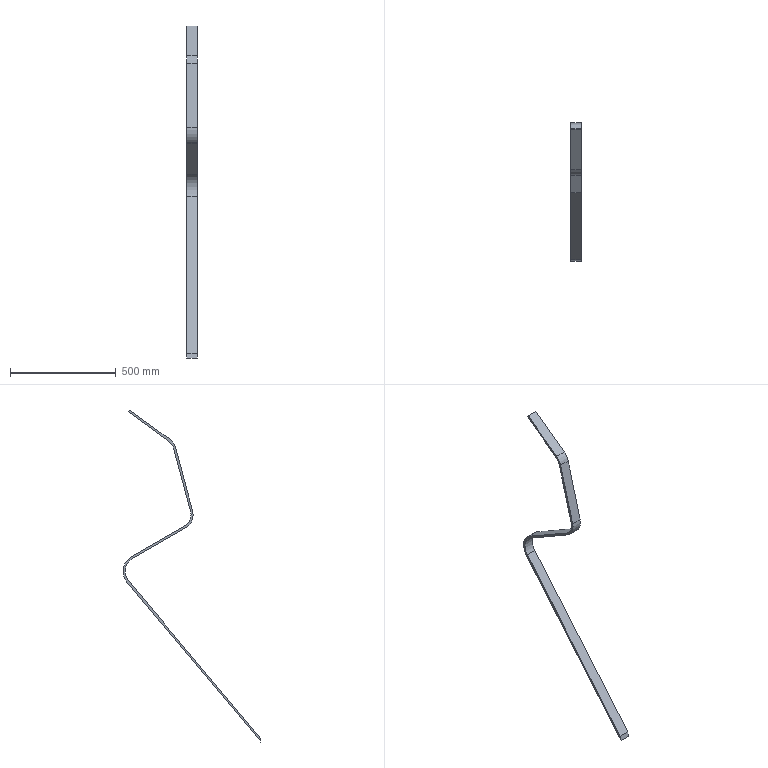Component | SolidWorks | Sipka resetke-1 | 1 solid | 20 faces | box 50 x 651.53 x 1567.49 mm | volume 1035206 mm3 | plane 12 | cylinder 8 | commonest cylinder face diameters 140 x4 120 x3 160 x1
STEP:
#1=COLOUR_RGB('',0.7922,0.8196,0.9333);
#2=FILL_AREA_STYLE_COLOUR('',#1);
#3=FILL_AREA_STYLE('',(#2));
#4=SURFACE_STYLE_FILL_AREA(#3);
#5=SURFACE_SIDE_STYLE('',(#4));
#6=SURFACE_STYLE_USAGE(.BOTH.,#5);
#7=PRESENTATION_STYLE_ASSIGNMENT((#6));
#8=CARTESIAN_POINT('',(-0.1417,16.681,-14.25));
#9=VERTEX_POINT('',#8);
#10=CARTESIAN_POINT('',(-0.1417,16.343,-14.014));
#11=VERTEX_POINT('',#10);
#12=CARTESIAN_POINT('',(-0.1417,17.861,-12.204));
#13=DIRECTION('',(-1.,0.,0.));
#14=DIRECTION('',(0.,0.6427,0.7661));
#15=AXIS2_PLACEMENT_3D('',#12,#13,#14);
#16=CIRCLE('',#15,2.362);
#17=EDGE_CURVE('',#9,#11,#16,.T.);
#18=ORIENTED_EDGE('',*,*,#17,.T.);
#19=CARTESIAN_POINT('',(1.827,16.343,-14.014));
#20=VERTEX_POINT('',#19);
#21=CARTESIAN_POINT('',(-0.1417,16.343,-14.014));
#22=DIRECTION('',(1.,-0.,-0.));
#23=VECTOR('',#22,39.37);
#24=LINE('',#21,#23);
#25=EDGE_CURVE('',#11,#20,#24,.T.);
#26=ORIENTED_EDGE('',*,*,#25,.T.);
#27=CARTESIAN_POINT('',(1.827,16.681,-14.25));
#28=VERTEX_POINT('',#27);
#29=CARTESIAN_POINT('',(1.827,17.861,-12.204));
#30=DIRECTION('',(-1.,0.,0.));
#31=DIRECTION('',(0.,0.6427,0.7661));
#32=AXIS2_PLACEMENT_3D('',#29,#30,#31);
#33=CIRCLE('',#32,2.362);
#34=EDGE_CURVE('',#28,#20,#33,.T.);
#35=ORIENTED_EDGE('',*,*,#34,.F.);
#36=CARTESIAN_POINT('',(-0.1417,16.681,-14.25));
#37=DIRECTION('',(1.,-0.,-0.));
#38=VECTOR('',#37,39.37);
#39=LINE('',#36,#38);
#40=EDGE_CURVE('',#9,#28,#39,.T.);
#41=ORIENTED_EDGE('',*,*,#40,.F.);
#42=EDGE_LOOP('',(#18,#26,#35,#41));
#43=FACE_OUTER_BOUND('',#42,.T.);
#44=CARTESIAN_POINT('',(-0.1417,17.861,-12.204));
#45=DIRECTION('',(1.,-0.,-0.));
#46=DIRECTION('',(-0.,-0.6427,-0.7661));
#47=AXIS2_PLACEMENT_3D('',#44,#45,#46);
#48=CYLINDRICAL_SURFACE('',#47,2.362);
#49=ADVANCED_FACE('',(#43),#48,.F.);
#50=CARTESIAN_POINT('',(-0.1417,15.199,-11.491));
#51=VERTEX_POINT('',#50);
#52=CARTESIAN_POINT('',(-0.1417,16.09,-14.315));
#53=VERTEX_POINT('',#52);
#54=CARTESIAN_POINT('',(-0.1417,17.861,-12.204));
#55=DIRECTION('',(1.,-0.,-0.));
#56=DIRECTION('',(0.,0.6427,0.7661));
#57=AXIS2_PLACEMENT_3D('',#54,#55,#56);
#58=CIRCLE('',#57,2.756);
#59=EDGE_CURVE('',#51,#53,#58,.T.);
#60=ORIENTED_EDGE('',*,*,#59,.T.);
#61=CARTESIAN_POINT('',(1.827,16.09,-14.315));
#62=VERTEX_POINT('',#61);
#63=CARTESIAN_POINT('',(-0.1417,16.09,-14.315));
#64=DIRECTION('',(1.,-0.,-0.));
#65=VECTOR('',#64,39.37);
#66=LINE('',#63,#65);
#67=EDGE_CURVE('',#53,#62,#66,.T.);
#68=ORIENTED_EDGE('',*,*,#67,.T.);
#69=CARTESIAN_POINT('',(1.827,15.199,-11.491));
#70=VERTEX_POINT('',#69);
#71=CARTESIAN_POINT('',(1.827,17.861,-12.204));
#72=DIRECTION('',(1.,-0.,-0.));
#73=DIRECTION('',(0.,0.6427,0.7661));
#74=AXIS2_PLACEMENT_3D('',#71,#72,#73);
#75=CIRCLE('',#74,2.756);
#76=EDGE_CURVE('',#70,#62,#75,.T.);
#77=ORIENTED_EDGE('',*,*,#76,.F.);
#78=CARTESIAN_POINT('',(-0.1417,15.199,-11.491));
#79=DIRECTION('',(1.,-0.,-0.));
#80=VECTOR('',#79,39.37);
#81=LINE('',#78,#80);
#82=EDGE_CURVE('',#51,#70,#81,.T.);
#83=ORIENTED_EDGE('',*,*,#82,.F.);
#84=EDGE_LOOP('',(#60,#68,#77,#83));
#85=FACE_OUTER_BOUND('',#84,.T.);
#86=CARTESIAN_POINT('',(-0.1417,17.861,-12.204));
#87=DIRECTION('',(1.,-0.,-0.));
#88=DIRECTION('',(-0.,-0.6427,-0.7661));
#89=AXIS2_PLACEMENT_3D('',#86,#87,#88);
#90=CYLINDRICAL_SURFACE('',#89,2.756);
#91=ADVANCED_FACE('',(#85),#90,.T.);
#92=CARTESIAN_POINT('',(-0.1417,2.493,-54.408));
#93=VERTEX_POINT('',#92);
#94=CARTESIAN_POINT('',(-0.1417,27.407,-24.709));
#95=VERTEX_POINT('',#94);
#96=CARTESIAN_POINT('',(-0.1417,2.104,-54.872));
#97=DIRECTION('',(0.,0.6427,0.7661));
#98=VECTOR('',#97,39.37);
#99=LINE('',#96,#98);
#100=EDGE_CURVE('',#93,#95,#99,.T.);
#101=ORIENTED_EDGE('',*,*,#100,.F.);
#102=CARTESIAN_POINT('',(-0.1417,2.705,-53.543));
#103=VERTEX_POINT('',#102);
#104=CARTESIAN_POINT('',(-0.1417,3.236,-51.372));
#105=DIRECTION('',(0.,0.2378,0.9713));
#106=VECTOR('',#105,39.37);
#107=LINE('',#104,#106);
#108=EDGE_CURVE('',#93,#103,#107,.T.);
#109=ORIENTED_EDGE('',*,*,#108,.T.);
#110=CARTESIAN_POINT('',(-0.1417,27.106,-24.456));
#111=VERTEX_POINT('',#110);
#112=CARTESIAN_POINT('',(-0.1417,1.803,-54.619));
#113=DIRECTION('',(-0.,-0.6427,-0.7661));
#114=VECTOR('',#113,39.37);
#115=LINE('',#112,#114);
#116=EDGE_CURVE('',#111,#103,#115,.T.);
#117=ORIENTED_EDGE('',*,*,#116,.F.);
#118=CARTESIAN_POINT('',(-0.1417,26.372,-20.298));
#119=VERTEX_POINT('',#118);
#120=CARTESIAN_POINT('',(-0.1417,24.994,-22.685));
#121=DIRECTION('',(-1.,0.,0.));
#122=DIRECTION('',(0.,0.6427,0.7661));
#123=AXIS2_PLACEMENT_3D('',#120,#121,#122);
#124=CIRCLE('',#123,2.756);
#125=EDGE_CURVE('',#119,#111,#124,.T.);
#126=ORIENTED_EDGE('',*,*,#125,.F.);
#127=CARTESIAN_POINT('',(-0.1417,16.484,-14.591));
#128=VERTEX_POINT('',#127);
#129=CARTESIAN_POINT('',(-0.1417,26.372,-20.298));
#130=DIRECTION('',(0.,0.8661,-0.4999));
#131=VECTOR('',#130,39.37);
#132=LINE('',#129,#131);
#133=EDGE_CURVE('',#128,#119,#132,.T.);
#134=ORIENTED_EDGE('',*,*,#133,.F.);
#135=CARTESIAN_POINT('',(-0.1417,17.861,-12.204));
#136=DIRECTION('',(1.,-0.,-0.));
#137=DIRECTION('',(0.,0.6427,0.7661));
#138=AXIS2_PLACEMENT_3D('',#135,#136,#137);
#139=CIRCLE('',#138,2.756);
#140=EDGE_CURVE('',#53,#128,#139,.T.);
#141=ORIENTED_EDGE('',*,*,#140,.F.);
#142=ORIENTED_EDGE('',*,*,#59,.F.);
#143=CARTESIAN_POINT('',(-0.1417,18.364,0.3205));
#144=VERTEX_POINT('',#143);
#145=CARTESIAN_POINT('',(-0.1417,15.199,-11.491));
#146=DIRECTION('',(-0.,-0.2588,-0.9659));
#147=VECTOR('',#146,39.37);
#148=LINE('',#145,#147);
#149=EDGE_CURVE('',#144,#51,#148,.T.);
#150=ORIENTED_EDGE('',*,*,#149,.F.);
#151=CARTESIAN_POINT('',(-0.1417,19.398,1.831));
#152=VERTEX_POINT('',#151);
#153=CARTESIAN_POINT('',(-0.1417,21.026,-0.3928));
#154=DIRECTION('',(1.,-0.,-0.));
#155=DIRECTION('',(-0.,-0.6427,-0.7661));
#156=AXIS2_PLACEMENT_3D('',#153,#154,#155);
#157=CIRCLE('',#156,2.756);
#158=EDGE_CURVE('',#152,#144,#157,.T.);
#159=ORIENTED_EDGE('',*,*,#158,.F.);
#160=CARTESIAN_POINT('',(-0.1417,26.874,7.304));
#161=VERTEX_POINT('',#160);
#162=CARTESIAN_POINT('',(-0.1417,19.398,1.831));
#163=DIRECTION('',(-0.,-0.8069,-0.5907));
#164=VECTOR('',#163,39.37);
#165=LINE('',#162,#164);
#166=EDGE_CURVE('',#161,#152,#165,.T.);
#167=ORIENTED_EDGE('',*,*,#166,.F.);
#168=CARTESIAN_POINT('',(-0.1417,27.107,6.987));
#169=VERTEX_POINT('',#168);
#170=CARTESIAN_POINT('',(-0.1417,27.107,6.987));
#171=DIRECTION('',(0.,-0.5907,0.8069));
#172=VECTOR('',#171,39.37);
#173=LINE('',#170,#172);
#174=EDGE_CURVE('',#169,#161,#173,.T.);
#175=ORIENTED_EDGE('',*,*,#174,.F.);
#176=CARTESIAN_POINT('',(-0.1417,19.631,1.513));
#177=VERTEX_POINT('',#176);
#178=CARTESIAN_POINT('',(-0.1417,19.631,1.513));
#179=DIRECTION('',(0.,0.8069,0.5907));
#180=VECTOR('',#179,39.37);
#181=LINE('',#178,#180);
#182=EDGE_CURVE('',#177,#169,#181,.T.);
#183=ORIENTED_EDGE('',*,*,#182,.F.);
#184=CARTESIAN_POINT('',(-0.1417,18.745,0.2186));
#185=VERTEX_POINT('',#184);
#186=CARTESIAN_POINT('',(-0.1417,21.026,-0.3928));
#187=DIRECTION('',(-1.,0.,0.));
#188=DIRECTION('',(-0.,-0.6427,-0.7661));
#189=AXIS2_PLACEMENT_3D('',#186,#187,#188);
#190=CIRCLE('',#189,2.362);
#191=EDGE_CURVE('',#185,#177,#190,.T.);
#192=ORIENTED_EDGE('',*,*,#191,.F.);
#193=CARTESIAN_POINT('',(-0.1417,15.58,-11.593));
#194=VERTEX_POINT('',#193);
#195=CARTESIAN_POINT('',(-0.1417,15.58,-11.593));
#196=DIRECTION('',(0.,0.2588,0.9659));
#197=VECTOR('',#196,39.37);
#198=LINE('',#195,#197);
#199=EDGE_CURVE('',#194,#185,#198,.T.);
#200=ORIENTED_EDGE('',*,*,#199,.F.);
#201=CARTESIAN_POINT('',(-0.1417,17.861,-12.204));
#202=DIRECTION('',(-1.,0.,0.));
#203=DIRECTION('',(0.,0.6427,0.7661));
#204=AXIS2_PLACEMENT_3D('',#201,#202,#203);
#205=CIRCLE('',#204,2.362);
#206=EDGE_CURVE('',#11,#194,#205,.T.);
#207=ORIENTED_EDGE('',*,*,#206,.F.);
#208=ORIENTED_EDGE('',*,*,#17,.F.);
#209=CARTESIAN_POINT('',(-0.1417,26.569,-19.957));
#210=VERTEX_POINT('',#209);
#211=CARTESIAN_POINT('',(-0.1417,26.569,-19.957));
#212=DIRECTION('',(-0.,-0.8661,0.4999));
#213=VECTOR('',#212,39.37);
#214=LINE('',#211,#213);
#215=EDGE_CURVE('',#210,#9,#214,.T.);
#216=ORIENTED_EDGE('',*,*,#215,.F.);
#217=CARTESIAN_POINT('',(-0.1417,24.994,-22.685));
#218=DIRECTION('',(1.,-0.,-0.));
#219=DIRECTION('',(0.,0.6427,0.7661));
#220=AXIS2_PLACEMENT_3D('',#217,#218,#219);
#221=CIRCLE('',#220,3.15);
#222=EDGE_CURVE('',#95,#210,#221,.T.);
#223=ORIENTED_EDGE('',*,*,#222,.F.);
#224=EDGE_LOOP('',(#101,#109,#117,#126,#134,#141,#142,#150,#159,#167,#175,#183,#192,#200,#207,#208,#216,#223));
#225=FACE_OUTER_BOUND('',#224,.T.);
#226=CARTESIAN_POINT('',(-0.1417,24.994,-22.685));
#227=DIRECTION('',(-1.,0.,0.));
#228=DIRECTION('',(0.,0.6427,0.7661));
#229=AXIS2_PLACEMENT_3D('',#226,#227,#228);
#230=PLANE('',#229);
#231=ADVANCED_FACE('',(#225),#230,.T.);
#232=CARTESIAN_POINT('',(1.827,2.493,-54.408));
#233=VERTEX_POINT('',#232);
#234=CARTESIAN_POINT('',(1.827,2.705,-53.543));
#235=VERTEX_POINT('',#234);
#236=CARTESIAN_POINT('',(1.827,3.236,-51.372));
#237=DIRECTION('',(0.,0.2378,0.9713));
#238=VECTOR('',#237,39.37);
#239=LINE('',#236,#238);
#240=EDGE_CURVE('',#233,#235,#239,.T.);
#241=ORIENTED_EDGE('',*,*,#240,.F.);
#242=CARTESIAN_POINT('',(1.827,27.407,-24.709));
#243=VERTEX_POINT('',#242);
#244=CARTESIAN_POINT('',(1.827,2.104,-54.872));
#245=DIRECTION('',(0.,0.6427,0.7661));
#246=VECTOR('',#245,39.37);
#247=LINE('',#244,#246);
#248=EDGE_CURVE('',#233,#243,#247,.T.);
#249=ORIENTED_EDGE('',*,*,#248,.T.);
#250=CARTESIAN_POINT('',(1.827,26.569,-19.957));
#251=VERTEX_POINT('',#250);
#252=CARTESIAN_POINT('',(1.827,24.994,-22.685));
#253=DIRECTION('',(1.,-0.,-0.));
#254=DIRECTION('',(0.,0.6427,0.7661));
#255=AXIS2_PLACEMENT_3D('',#252,#253,#254);
#256=CIRCLE('',#255,3.15);
#257=EDGE_CURVE('',#243,#251,#256,.T.);
#258=ORIENTED_EDGE('',*,*,#257,.T.);
#259=CARTESIAN_POINT('',(1.827,26.569,-19.957));
#260=DIRECTION('',(-0.,-0.8661,0.4999));
#261=VECTOR('',#260,39.37);
#262=LINE('',#259,#261);
#263=EDGE_CURVE('',#251,#28,#262,.T.);
#264=ORIENTED_EDGE('',*,*,#263,.T.);
#265=ORIENTED_EDGE('',*,*,#34,.T.);
#266=CARTESIAN_POINT('',(1.827,15.58,-11.593));
#267=VERTEX_POINT('',#266);
#268=CARTESIAN_POINT('',(1.827,17.861,-12.204));
#269=DIRECTION('',(-1.,0.,0.));
#270=DIRECTION('',(0.,0.6427,0.7661));
#271=AXIS2_PLACEMENT_3D('',#268,#269,#270);
#272=CIRCLE('',#271,2.362);
#273=EDGE_CURVE('',#20,#267,#272,.T.);
#274=ORIENTED_EDGE('',*,*,#273,.T.);
#275=CARTESIAN_POINT('',(1.827,18.745,0.2186));
#276=VERTEX_POINT('',#275);
#277=CARTESIAN_POINT('',(1.827,15.58,-11.593));
#278=DIRECTION('',(0.,0.2588,0.9659));
#279=VECTOR('',#278,39.37);
#280=LINE('',#277,#279);
#281=EDGE_CURVE('',#267,#276,#280,.T.);
#282=ORIENTED_EDGE('',*,*,#281,.T.);
#283=CARTESIAN_POINT('',(1.827,19.631,1.513));
#284=VERTEX_POINT('',#283);
#285=CARTESIAN_POINT('',(1.827,21.026,-0.3928));
#286=DIRECTION('',(-1.,0.,0.));
#287=DIRECTION('',(0.,-0.6427,-0.7661));
#288=AXIS2_PLACEMENT_3D('',#285,#286,#287);
#289=CIRCLE('',#288,2.362);
#290=EDGE_CURVE('',#276,#284,#289,.T.);
#291=ORIENTED_EDGE('',*,*,#290,.T.);
#292=CARTESIAN_POINT('',(1.827,27.107,6.987));
#293=VERTEX_POINT('',#292);
#294=CARTESIAN_POINT('',(1.827,19.631,1.513));
#295=DIRECTION('',(0.,0.8069,0.5907));
#296=VECTOR('',#295,39.37);
#297=LINE('',#294,#296);
#298=EDGE_CURVE('',#284,#293,#297,.T.);
#299=ORIENTED_EDGE('',*,*,#298,.T.);
#300=CARTESIAN_POINT('',(1.827,26.874,7.304));
#301=VERTEX_POINT('',#300);
#302=CARTESIAN_POINT('',(1.827,27.107,6.987));
#303=DIRECTION('',(0.,-0.5907,0.8069));
#304=VECTOR('',#303,39.37);
#305=LINE('',#302,#304);
#306=EDGE_CURVE('',#293,#301,#305,.T.);
#307=ORIENTED_EDGE('',*,*,#306,.T.);
#308=CARTESIAN_POINT('',(1.827,19.398,1.831));
#309=VERTEX_POINT('',#308);
#310=CARTESIAN_POINT('',(1.827,19.398,1.831));
#311=DIRECTION('',(-0.,-0.8069,-0.5907));
#312=VECTOR('',#311,39.37);
#313=LINE('',#310,#312);
#314=EDGE_CURVE('',#301,#309,#313,.T.);
#315=ORIENTED_EDGE('',*,*,#314,.T.);
#316=CARTESIAN_POINT('',(1.827,18.364,0.3205));
#317=VERTEX_POINT('',#316);
#318=CARTESIAN_POINT('',(1.827,21.026,-0.3928));
#319=DIRECTION('',(1.,-0.,-0.));
#320=DIRECTION('',(0.,-0.6427,-0.7661));
#321=AXIS2_PLACEMENT_3D('',#318,#319,#320);
#322=CIRCLE('',#321,2.756);
#323=EDGE_CURVE('',#309,#317,#322,.T.);
#324=ORIENTED_EDGE('',*,*,#323,.T.);
#325=CARTESIAN_POINT('',(1.827,15.199,-11.491));
#326=DIRECTION('',(-0.,-0.2588,-0.9659));
#327=VECTOR('',#326,39.37);
#328=LINE('',#325,#327);
#329=EDGE_CURVE('',#317,#70,#328,.T.);
#330=ORIENTED_EDGE('',*,*,#329,.T.);
#331=ORIENTED_EDGE('',*,*,#76,.T.);
#332=CARTESIAN_POINT('',(1.827,16.484,-14.591));
#333=VERTEX_POINT('',#332);
#334=CARTESIAN_POINT('',(1.827,17.861,-12.204));
#335=DIRECTION('',(1.,-0.,-0.));
#336=DIRECTION('',(0.,0.6427,0.7661));
#337=AXIS2_PLACEMENT_3D('',#334,#335,#336);
#338=CIRCLE('',#337,2.756);
#339=EDGE_CURVE('',#62,#333,#338,.T.);
#340=ORIENTED_EDGE('',*,*,#339,.T.);
#341=CARTESIAN_POINT('',(1.827,26.372,-20.298));
#342=VERTEX_POINT('',#341);
#343=CARTESIAN_POINT('',(1.827,26.372,-20.298));
#344=DIRECTION('',(0.,0.8661,-0.4999));
#345=VECTOR('',#344,39.37);
#346=LINE('',#343,#345);
#347=EDGE_CURVE('',#333,#342,#346,.T.);
#348=ORIENTED_EDGE('',*,*,#347,.T.);
#349=CARTESIAN_POINT('',(1.827,27.106,-24.456));
#350=VERTEX_POINT('',#349);
#351=CARTESIAN_POINT('',(1.827,24.994,-22.685));
#352=DIRECTION('',(-1.,0.,0.));
#353=DIRECTION('',(0.,0.6427,0.7661));
#354=AXIS2_PLACEMENT_3D('',#351,#352,#353);
#355=CIRCLE('',#354,2.756);
#356=EDGE_CURVE('',#342,#350,#355,.T.);
#357=ORIENTED_EDGE('',*,*,#356,.T.);
#358=CARTESIAN_POINT('',(1.827,1.803,-54.619));
#359=DIRECTION('',(-0.,-0.6427,-0.7661));
#360=VECTOR('',#359,39.37);
#361=LINE('',#358,#360);
#362=EDGE_CURVE('',#350,#235,#361,.T.);
#363=ORIENTED_EDGE('',*,*,#362,.T.);
#364=EDGE_LOOP('',(#241,#249,#258,#264,#265,#274,#282,#291,#299,#307,#315,#324,#330,#331,#340,#348,#357,#363));
#365=FACE_OUTER_BOUND('',#364,.T.);
#366=CARTESIAN_POINT('',(1.827,24.994,-22.685));
#367=DIRECTION('',(-1.,0.,0.));
#368=DIRECTION('',(0.,0.6427,0.7661));
#369=AXIS2_PLACEMENT_3D('',#366,#367,#368);
#370=PLANE('',#369);
#371=ADVANCED_FACE('',(#365),#370,.F.);
#372=CARTESIAN_POINT('',(-0.1417,2.705,-53.543));
#373=DIRECTION('',(-1.,0.,0.));
#374=VECTOR('',#373,39.37);
#375=LINE('',#372,#374);
#376=EDGE_CURVE('',#235,#103,#375,.T.);
#377=ORIENTED_EDGE('',*,*,#376,.F.);
#378=ORIENTED_EDGE('',*,*,#362,.F.);
#379=CARTESIAN_POINT('',(-0.1417,27.106,-24.456));
#380=DIRECTION('',(1.,-0.,-0.));
#381=VECTOR('',#380,39.37);
#382=LINE('',#379,#381);
#383=EDGE_CURVE('',#111,#350,#382,.T.);
#384=ORIENTED_EDGE('',*,*,#383,.F.);
#385=ORIENTED_EDGE('',*,*,#116,.T.);
#386=EDGE_LOOP('',(#377,#378,#384,#385));
#387=FACE_OUTER_BOUND('',#386,.T.);
#388=CARTESIAN_POINT('',(-0.1417,1.803,-54.619));
#389=DIRECTION('',(-0.,-0.7661,0.6427));
#390=DIRECTION('',(-0.,-0.6427,-0.7661));
#391=AXIS2_PLACEMENT_3D('',#388,#389,#390);
#392=PLANE('',#391);
#393=ADVANCED_FACE('',(#387),#392,.T.);
#394=ORIENTED_EDGE('',*,*,#356,.F.);
#395=CARTESIAN_POINT('',(-0.1417,26.372,-20.298));
#396=DIRECTION('',(1.,-0.,-0.));
#397=VECTOR('',#396,39.37);
#398=LINE('',#395,#397);
#399=EDGE_CURVE('',#119,#342,#398,.T.);
#400=ORIENTED_EDGE('',*,*,#399,.F.);
#401=ORIENTED_EDGE('',*,*,#125,.T.);
#402=ORIENTED_EDGE('',*,*,#383,.T.);
#403=EDGE_LOOP('',(#394,#400,#401,#402));
#404=FACE_OUTER_BOUND('',#403,.T.);
#405=CARTESIAN_POINT('',(-0.1417,24.994,-22.685));
#406=DIRECTION('',(1.,-0.,-0.));
#407=DIRECTION('',(-0.,-0.6427,-0.7661));
#408=AXIS2_PLACEMENT_3D('',#405,#406,#407);
#409=CYLINDRICAL_SURFACE('',#408,2.756);
#410=ADVANCED_FACE('',(#404),#409,.F.);
#411=ORIENTED_EDGE('',*,*,#347,.F.);
#412=CARTESIAN_POINT('',(-0.1417,16.484,-14.591));
#413=DIRECTION('',(1.,-0.,-0.));
#414=VECTOR('',#413,39.37);
#415=LINE('',#412,#414);
#416=EDGE_CURVE('',#128,#333,#415,.T.);
#417=ORIENTED_EDGE('',*,*,#416,.F.);
#418=ORIENTED_EDGE('',*,*,#133,.T.);
#419=ORIENTED_EDGE('',*,*,#399,.T.);
#420=EDGE_LOOP('',(#411,#417,#418,#419));
#421=FACE_OUTER_BOUND('',#420,.T.);
#422=CARTESIAN_POINT('',(-0.1417,26.372,-20.298));
#423=DIRECTION('',(-0.,-0.4999,-0.8661));
#424=DIRECTION('',(0.,0.8661,-0.4999));
#425=AXIS2_PLACEMENT_3D('',#422,#423,#424);
#426=PLANE('',#425);
#427=ADVANCED_FACE('',(#421),#426,.T.);
#428=ORIENTED_EDGE('',*,*,#67,.F.);
#429=ORIENTED_EDGE('',*,*,#140,.T.);
#430=ORIENTED_EDGE('',*,*,#416,.T.);
#431=ORIENTED_EDGE('',*,*,#339,.F.);
#432=EDGE_LOOP('',(#428,#429,#430,#431));
#433=FACE_OUTER_BOUND('',#432,.T.);
#434=CARTESIAN_POINT('',(-0.1417,17.861,-12.204));
#435=DIRECTION('',(1.,-0.,-0.));
#436=DIRECTION('',(-0.,-0.6427,-0.7661));
#437=AXIS2_PLACEMENT_3D('',#434,#435,#436);
#438=CYLINDRICAL_SURFACE('',#437,2.756);
#439=ADVANCED_FACE('',(#433),#438,.T.);
#440=ORIENTED_EDGE('',*,*,#329,.F.);
#441=CARTESIAN_POINT('',(-0.1417,18.364,0.3205));
#442=DIRECTION('',(1.,-0.,-0.));
#443=VECTOR('',#442,39.37);
#444=LINE('',#441,#443);
#445=EDGE_CURVE('',#144,#317,#444,.T.);
#446=ORIENTED_EDGE('',*,*,#445,.F.);
#447=ORIENTED_EDGE('',*,*,#149,.T.);
#448=ORIENTED_EDGE('',*,*,#82,.T.);
#449=EDGE_LOOP('',(#440,#446,#447,#448));
#450=FACE_OUTER_BOUND('',#449,.T.);
#451=CARTESIAN_POINT('',(-0.1417,15.199,-11.491));
#452=DIRECTION('',(-0.,-0.9659,0.2588));
#453=DIRECTION('',(-0.,-0.2588,-0.9659));
#454=AXIS2_PLACEMENT_3D('',#451,#452,#453);
#455=PLANE('',#454);
#456=ADVANCED_FACE('',(#450),#455,.T.);
#457=ORIENTED_EDGE('',*,*,#323,.F.);
#458=CARTESIAN_POINT('',(-0.1417,19.398,1.831));
#459=DIRECTION('',(1.,-0.,-0.));
#460=VECTOR('',#459,39.37);
#461=LINE('',#458,#460);
#462=EDGE_CURVE('',#152,#309,#461,.T.);
#463=ORIENTED_EDGE('',*,*,#462,.F.);
#464=ORIENTED_EDGE('',*,*,#158,.T.);
#465=ORIENTED_EDGE('',*,*,#445,.T.);
#466=EDGE_LOOP('',(#457,#463,#464,#465));
#467=FACE_OUTER_BOUND('',#466,.T.);
#468=CARTESIAN_POINT('',(-0.1417,21.026,-0.3928));
#469=DIRECTION('',(1.,-0.,-0.));
#470=DIRECTION('',(-0.,-0.6427,-0.7661));
#471=AXIS2_PLACEMENT_3D('',#468,#469,#470);
#472=CYLINDRICAL_SURFACE('',#471,2.756);
#473=ADVANCED_FACE('',(#467),#472,.T.);
#474=ORIENTED_EDGE('',*,*,#314,.F.);
#475=CARTESIAN_POINT('',(-0.1417,26.874,7.304));
#476=DIRECTION('',(1.,-0.,-0.));
#477=VECTOR('',#476,39.37);
#478=LINE('',#475,#477);
#479=EDGE_CURVE('',#161,#301,#478,.T.);
#480=ORIENTED_EDGE('',*,*,#479,.F.);
#481=ORIENTED_EDGE('',*,*,#166,.T.);
#482=ORIENTED_EDGE('',*,*,#462,.T.);
#483=EDGE_LOOP('',(#474,#480,#481,#482));
#484=FACE_OUTER_BOUND('',#483,.T.);
#485=CARTESIAN_POINT('',(-0.1417,19.398,1.831));
#486=DIRECTION('',(0.,-0.5907,0.8069));
#487=DIRECTION('',(-0.,-0.8069,-0.5907));
#488=AXIS2_PLACEMENT_3D('',#485,#486,#487);
#489=PLANE('',#488);
#490=ADVANCED_FACE('',(#484),#489,.T.);
#491=ORIENTED_EDGE('',*,*,#306,.F.);
#492=CARTESIAN_POINT('',(-0.1417,27.107,6.987));
#493=DIRECTION('',(1.,-0.,-0.));
#494=VECTOR('',#493,39.37);
#495=LINE('',#492,#494);
#496=EDGE_CURVE('',#169,#293,#495,.T.);
#497=ORIENTED_EDGE('',*,*,#496,.F.);
#498=ORIENTED_EDGE('',*,*,#174,.T.);
#499=ORIENTED_EDGE('',*,*,#479,.T.);
#500=EDGE_LOOP('',(#491,#497,#498,#499));
#501=FACE_OUTER_BOUND('',#500,.T.);
#502=CARTESIAN_POINT('',(-0.1417,27.107,6.987));
#503=DIRECTION('',(0.,0.8069,0.5907));
#504=DIRECTION('',(0.,-0.5907,0.8069));
#505=AXIS2_PLACEMENT_3D('',#502,#503,#504);
#506=PLANE('',#505);
#507=ADVANCED_FACE('',(#501),#506,.T.);
#508=ORIENTED_EDGE('',*,*,#298,.F.);
#509=CARTESIAN_POINT('',(-0.1417,19.631,1.513));
#510=DIRECTION('',(1.,-0.,-0.));
#511=VECTOR('',#510,39.37);
#512=LINE('',#509,#511);
#513=EDGE_CURVE('',#177,#284,#512,.T.);
#514=ORIENTED_EDGE('',*,*,#513,.F.);
#515=ORIENTED_EDGE('',*,*,#182,.T.);
#516=ORIENTED_EDGE('',*,*,#496,.T.);
#517=EDGE_LOOP('',(#508,#514,#515,#516));
#518=FACE_OUTER_BOUND('',#517,.T.);
#519=CARTESIAN_POINT('',(-0.1417,19.631,1.513));
#520=DIRECTION('',(-0.,0.5907,-0.8069));
#521=DIRECTION('',(0.,0.8069,0.5907));
#522=AXIS2_PLACEMENT_3D('',#519,#520,#521);
#523=PLANE('',#522);
#524=ADVANCED_FACE('',(#518),#523,.T.);
#525=ORIENTED_EDGE('',*,*,#290,.F.);
#526=CARTESIAN_POINT('',(-0.1417,18.745,0.2186));
#527=DIRECTION('',(1.,-0.,-0.));
#528=VECTOR('',#527,39.37);
#529=LINE('',#526,#528);
#530=EDGE_CURVE('',#185,#276,#529,.T.);
#531=ORIENTED_EDGE('',*,*,#530,.F.);
#532=ORIENTED_EDGE('',*,*,#191,.T.);
#533=ORIENTED_EDGE('',*,*,#513,.T.);
#534=EDGE_LOOP('',(#525,#531,#532,#533));
#535=FACE_OUTER_BOUND('',#534,.T.);
#536=CARTESIAN_POINT('',(-0.1417,21.026,-0.3928));
#537=DIRECTION('',(1.,-0.,-0.));
#538=DIRECTION('',(-0.,-0.6427,-0.7661));
#539=AXIS2_PLACEMENT_3D('',#536,#537,#538);
#540=CYLINDRICAL_SURFACE('',#539,2.362);
#541=ADVANCED_FACE('',(#535),#540,.F.);
#542=ORIENTED_EDGE('',*,*,#281,.F.);
#543=CARTESIAN_POINT('',(-0.1417,15.58,-11.593));
#544=DIRECTION('',(1.,-0.,-0.));
#545=VECTOR('',#544,39.37);
#546=LINE('',#543,#545);
#547=EDGE_CURVE('',#194,#267,#546,.T.);
#548=ORIENTED_EDGE('',*,*,#547,.F.);
#549=ORIENTED_EDGE('',*,*,#199,.T.);
#550=ORIENTED_EDGE('',*,*,#530,.T.);
#551=EDGE_LOOP('',(#542,#548,#549,#550));
#552=FACE_OUTER_BOUND('',#551,.T.);
#553=CARTESIAN_POINT('',(-0.1417,15.58,-11.593));
#554=DIRECTION('',(0.,0.9659,-0.2588));
#555=DIRECTION('',(0.,0.2588,0.9659));
#556=AXIS2_PLACEMENT_3D('',#553,#554,#555);
#557=PLANE('',#556);
#558=ADVANCED_FACE('',(#552),#557,.T.);
#559=ORIENTED_EDGE('',*,*,#25,.F.);
#560=ORIENTED_EDGE('',*,*,#206,.T.);
#561=ORIENTED_EDGE('',*,*,#547,.T.);
#562=ORIENTED_EDGE('',*,*,#273,.F.);
#563=EDGE_LOOP('',(#559,#560,#561,#562));
#564=FACE_OUTER_BOUND('',#563,.T.);
#565=CARTESIAN_POINT('',(-0.1417,17.861,-12.204));
#566=DIRECTION('',(1.,-0.,-0.));
#567=DIRECTION('',(-0.,-0.6427,-0.7661));
#568=AXIS2_PLACEMENT_3D('',#565,#566,#567);
#569=CYLINDRICAL_SURFACE('',#568,2.362);
#570=ADVANCED_FACE('',(#564),#569,.F.);
#571=ORIENTED_EDGE('',*,*,#263,.F.);
#572=CARTESIAN_POINT('',(-0.1417,26.569,-19.957));
#573=DIRECTION('',(1.,-0.,-0.));
#574=VECTOR('',#573,39.37);
#575=LINE('',#572,#574);
#576=EDGE_CURVE('',#210,#251,#575,.T.);
#577=ORIENTED_EDGE('',*,*,#576,.F.);
#578=ORIENTED_EDGE('',*,*,#215,.T.);
#579=ORIENTED_EDGE('',*,*,#40,.T.);
#580=EDGE_LOOP('',(#571,#577,#578,#579));
#581=FACE_OUTER_BOUND('',#580,.T.);
#582=CARTESIAN_POINT('',(-0.1417,26.569,-19.957));
#583=DIRECTION('',(0.,0.4999,0.8661));
#584=DIRECTION('',(-0.,-0.8661,0.4999));
#585=AXIS2_PLACEMENT_3D('',#582,#583,#584);
#586=PLANE('',#585);
#587=ADVANCED_FACE('',(#581),#586,.T.);
#588=ORIENTED_EDGE('',*,*,#257,.F.);
#589=CARTESIAN_POINT('',(-0.1417,27.407,-24.709));
#590=DIRECTION('',(1.,-0.,-0.));
#591=VECTOR('',#590,39.37);
#592=LINE('',#589,#591);
#593=EDGE_CURVE('',#95,#243,#592,.T.);
#594=ORIENTED_EDGE('',*,*,#593,.F.);
#595=ORIENTED_EDGE('',*,*,#222,.T.);
#596=ORIENTED_EDGE('',*,*,#576,.T.);
#597=EDGE_LOOP('',(#588,#594,#595,#596));
#598=FACE_OUTER_BOUND('',#597,.T.);
#599=CARTESIAN_POINT('',(-0.1417,24.994,-22.685));
#600=DIRECTION('',(1.,-0.,-0.));
#601=DIRECTION('',(-0.,-0.6427,-0.7661));
#602=AXIS2_PLACEMENT_3D('',#599,#600,#601);
#603=CYLINDRICAL_SURFACE('',#602,3.15);
#604=ADVANCED_FACE('',(#598),#603,.T.);
#605=CARTESIAN_POINT('',(-0.1417,2.493,-54.408));
#606=DIRECTION('',(1.,-0.,-0.));
#607=VECTOR('',#606,39.37);
#608=LINE('',#605,#607);
#609=EDGE_CURVE('',#93,#233,#608,.T.);
#610=ORIENTED_EDGE('',*,*,#609,.F.);
#611=ORIENTED_EDGE('',*,*,#100,.T.);
#612=ORIENTED_EDGE('',*,*,#593,.T.);
#613=ORIENTED_EDGE('',*,*,#248,.F.);
#614=EDGE_LOOP('',(#610,#611,#612,#613));
#615=FACE_OUTER_BOUND('',#614,.T.);
#616=CARTESIAN_POINT('',(-0.1417,2.104,-54.872));
#617=DIRECTION('',(0.,0.7661,-0.6427));
#618=DIRECTION('',(1.,-0.,-0.));
#619=AXIS2_PLACEMENT_3D('',#616,#617,#618);
#620=PLANE('',#619);
#621=ADVANCED_FACE('',(#615),#620,.T.);
#622=ORIENTED_EDGE('',*,*,#376,.T.);
#623=ORIENTED_EDGE('',*,*,#108,.F.);
#624=ORIENTED_EDGE('',*,*,#609,.T.);
#625=ORIENTED_EDGE('',*,*,#240,.T.);
#626=EDGE_LOOP('',(#622,#623,#624,#625));
#627=FACE_OUTER_BOUND('',#626,.T.);
#628=CARTESIAN_POINT('',(-0.1417,3.236,-51.372));
#629=DIRECTION('',(0.,0.9713,-0.2378));
#630=DIRECTION('',(0.,0.2378,0.9713));
#631=AXIS2_PLACEMENT_3D('',#628,#629,#630);
#632=PLANE('',#631);
#633=ADVANCED_FACE('',(#627),#632,.F.);
#634=CLOSED_SHELL('',(#49,#91,#231,#371,#393,#410,#427,#439,#456,#473,#490,#507,#524,#541,#558,#570,#587,#604,#621,#633));
#635=MANIFOLD_SOLID_BREP('',#634);
#636=STYLED_ITEM('',(#7),#635);
#637=(LENGTH_UNIT()NAMED_UNIT(*)SI_UNIT($,.METRE.));
#638=LENGTH_MEASURE_WITH_UNIT(LENGTH_MEASURE(0.0254),#637);
#639=DIMENSIONAL_EXPONENTS(1.,0.,0.,0.,0.,0.,0.);
#640=(CONVERSION_BASED_UNIT('',#638)LENGTH_UNIT()NAMED_UNIT(#639));
#641=UNCERTAINTY_MEASURE_WITH_UNIT(LENGTH_MEASURE(0.00001),#640,'','');
#642=(NAMED_UNIT(*)PLANE_ANGLE_UNIT()SI_UNIT($,.RADIAN.));
#643=(NAMED_UNIT(*)SI_UNIT($,.STERADIAN.)SOLID_ANGLE_UNIT());
#644=(GEOMETRIC_REPRESENTATION_CONTEXT(3)GLOBAL_UNCERTAINTY_ASSIGNED_CONTEXT((#641))GLOBAL_UNIT_ASSIGNED_CONTEXT((#640,#642,#643))REPRESENTATION_CONTEXT('',''));
#645=MECHANICAL_DESIGN_GEOMETRIC_PRESENTATION_REPRESENTATION('',(#636),#644);
#646=PRESENTATION_LAYER_ASSIGNMENT('','',(#636));
#647=CARTESIAN_POINT('',(0.,0.,0.));
#648=DIRECTION('',(0.,0.,1.));
#649=DIRECTION('',(1.,0.,0.));
#650=AXIS2_PLACEMENT_3D('',#647,#648,#649);
#651=(LENGTH_UNIT()NAMED_UNIT(*)SI_UNIT($,.METRE.));
#652=LENGTH_MEASURE_WITH_UNIT(LENGTH_MEASURE(0.0254),#651);
#653=DIMENSIONAL_EXPONENTS(1.,0.,0.,0.,0.,0.,0.);
#654=(CONVERSION_BASED_UNIT('',#652)LENGTH_UNIT()NAMED_UNIT(#653));
#655=UNCERTAINTY_MEASURE_WITH_UNIT(LENGTH_MEASURE(0.00001),#654,'','');
#656=(NAMED_UNIT(*)PLANE_ANGLE_UNIT()SI_UNIT($,.RADIAN.));
#657=(NAMED_UNIT(*)SI_UNIT($,.STERADIAN.)SOLID_ANGLE_UNIT());
#658=(GEOMETRIC_REPRESENTATION_CONTEXT(3)GLOBAL_UNCERTAINTY_ASSIGNED_CONTEXT((#655))GLOBAL_UNIT_ASSIGNED_CONTEXT((#654,#656,#657))REPRESENTATION_CONTEXT('',''));
#659=ADVANCED_BREP_SHAPE_REPRESENTATION('',(#635,#650),#658);